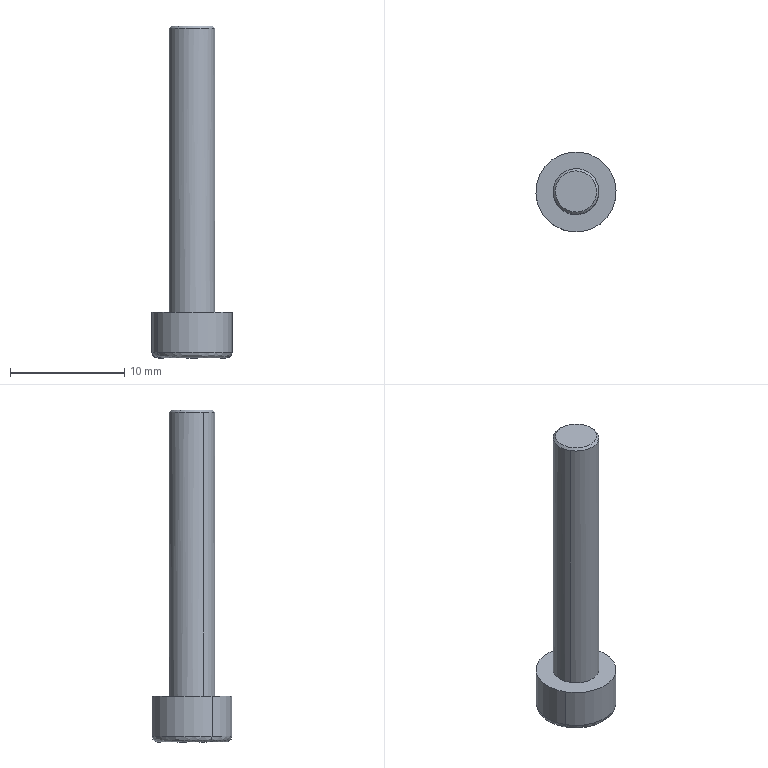Component | SolidWorks | M4X25-5 | 1 solid | 25 faces | box 7 x 7 x 29 mm | volume 449 mm3 | plane 15 | cylinder 4 | cone 4 | spline 2 | commonest cylinder face diameters 4 x2 7 x2 | material Standard Part
STEP:
#1=CARTESIAN_POINT('',(-0.7212,0.5163,-1.24));
#2=VERTEX_POINT('',#1);
#3=CARTESIAN_POINT('',(-0.9599,0.3785,-1.24));
#4=VERTEX_POINT('',#3);
#5=CARTESIAN_POINT('',(-0.8406,0.4474,-1.24));
#6=DIRECTION('',(-0.,-0.,1.));
#7=DIRECTION('',(0.866,0.5,0.));
#8=AXIS2_PLACEMENT_3D('',#5,#6,#7);
#9=CIRCLE('',#8,0.1378);
#10=EDGE_CURVE('',#2,#4,#9,.T.);
#11=ORIENTED_EDGE('',*,*,#10,.F.);
#12=CARTESIAN_POINT('',(-0.7383,0.5065,-1.26));
#13=VERTEX_POINT('',#12);
#14=CARTESIAN_POINT('',(-0.7383,0.5065,-1.24));
#15=DIRECTION('',(-0.5,0.866,-0.));
#16=DIRECTION('',(0.866,0.5,0.));
#17=AXIS2_PLACEMENT_3D('',#14,#15,#16);
#18=CIRCLE('',#17,0.01969);
#19=EDGE_CURVE('',#2,#13,#18,.T.);
#20=ORIENTED_EDGE('',*,*,#19,.T.);
#21=CARTESIAN_POINT('',(-0.9429,0.3884,-1.26));
#22=VERTEX_POINT('',#21);
#23=CARTESIAN_POINT('',(-0.7383,0.5065,-1.26));
#24=CARTESIAN_POINT('',(-0.8564,0.711,-1.26));
#25=CARTESIAN_POINT('',(-1.061,0.5929,-1.26));
#26=CARTESIAN_POINT('',(-0.9429,0.3884,-1.26));
#27=(BOUNDED_CURVE()B_SPLINE_CURVE(3,(#23,#24,#25,#26),.UNSPECIFIED.,.F.,.T.)B_SPLINE_CURVE_WITH_KNOTS((4,4),(0.,1.),.UNSPECIFIED.)CURVE()GEOMETRIC_REPRESENTATION_ITEM()RATIONAL_B_SPLINE_CURVE((1.,0.3333,0.3333,1.))REPRESENTATION_ITEM(''));
#28=EDGE_CURVE('',#13,#22,#27,.T.);
#29=ORIENTED_EDGE('',*,*,#28,.T.);
#30=CARTESIAN_POINT('',(-0.9429,0.3884,-1.24));
#31=DIRECTION('',(0.5,-0.866,0.));
#32=DIRECTION('',(-0.866,-0.5,0.));
#33=AXIS2_PLACEMENT_3D('',#30,#31,#32);
#34=CIRCLE('',#33,0.01969);
#35=EDGE_CURVE('',#4,#22,#34,.T.);
#36=ORIENTED_EDGE('',*,*,#35,.F.);
#37=EDGE_LOOP('',(#11,#20,#29,#36));
#38=FACE_OUTER_BOUND('',#37,.T.);
#39=CARTESIAN_POINT('',(-0.7212,0.5163,-1.24));
#40=CARTESIAN_POINT('',(-0.859,0.755,-1.24));
#41=CARTESIAN_POINT('',(-1.098,0.6172,-1.24));
#42=CARTESIAN_POINT('',(-0.9599,0.3785,-1.24));
#43=CARTESIAN_POINT('',(-0.7212,0.5163,-1.252));
#44=CARTESIAN_POINT('',(-0.859,0.755,-1.252));
#45=CARTESIAN_POINT('',(-1.098,0.6172,-1.252));
#46=CARTESIAN_POINT('',(-0.9599,0.3785,-1.252));
#47=CARTESIAN_POINT('',(-0.7283,0.5122,-1.26));
#48=CARTESIAN_POINT('',(-0.858,0.7368,-1.26));
#49=CARTESIAN_POINT('',(-1.082,0.6071,-1.26));
#50=CARTESIAN_POINT('',(-0.9529,0.3826,-1.26));
#51=CARTESIAN_POINT('',(-0.7383,0.5065,-1.26));
#52=CARTESIAN_POINT('',(-0.8564,0.711,-1.26));
#53=CARTESIAN_POINT('',(-1.061,0.5929,-1.26));
#54=CARTESIAN_POINT('',(-0.9429,0.3884,-1.26));
#55=(BOUNDED_SURFACE()B_SPLINE_SURFACE(3,3,((#39,#40,#41,#42),(#43,#44,#45,#46),(#47,#48,#49,#50),(#51,#52,#53,#54)),.UNSPECIFIED.,.F.,.F.,.F.)B_SPLINE_SURFACE_WITH_KNOTS((4,4),(4,4),(0.,1.),(0.,1.),.UNSPECIFIED.)GEOMETRIC_REPRESENTATION_ITEM()RATIONAL_B_SPLINE_SURFACE(((1.,0.3333,0.3333,1.),(0.8047,0.2682,0.2682,0.8047),(0.8047,0.2682,0.2682,0.8047),(1.,0.3333,0.3333,1.)))REPRESENTATION_ITEM('')SURFACE());
#56=ADVANCED_FACE('',(#38),#55,.T.);
#57=CARTESIAN_POINT('',(-0.8012,0.3792,-0.126));
#58=VERTEX_POINT('',#57);
#59=CARTESIAN_POINT('',(-0.9088,0.408,-0.126));
#60=VERTEX_POINT('',#59);
#61=CARTESIAN_POINT('',(-0.8406,0.4474,-0.126));
#62=DIRECTION('',(0.,0.,-1.));
#63=DIRECTION('',(0.866,0.5,0.));
#64=AXIS2_PLACEMENT_3D('',#61,#62,#63);
#65=CIRCLE('',#64,0.07874);
#66=EDGE_CURVE('',#58,#60,#65,.T.);
#67=ORIENTED_EDGE('',*,*,#66,.T.);
#68=CARTESIAN_POINT('',(-0.9088,0.408,-1.102));
#69=VERTEX_POINT('',#68);
#70=CARTESIAN_POINT('',(-0.9088,0.408,-0.1181));
#71=DIRECTION('',(0.,0.,-1.));
#72=VECTOR('',#71,39.37);
#73=LINE('',#70,#72);
#74=EDGE_CURVE('',#60,#69,#73,.T.);
#75=ORIENTED_EDGE('',*,*,#74,.T.);
#76=CARTESIAN_POINT('',(-0.7724,0.4868,-1.102));
#77=VERTEX_POINT('',#76);
#78=CARTESIAN_POINT('',(-0.8406,0.4474,-1.102));
#79=DIRECTION('',(-0.,-0.,1.));
#80=DIRECTION('',(0.866,0.5,0.));
#81=AXIS2_PLACEMENT_3D('',#78,#79,#80);
#82=CIRCLE('',#81,0.07874);
#83=EDGE_CURVE('',#69,#77,#82,.T.);
#84=ORIENTED_EDGE('',*,*,#83,.T.);
#85=CARTESIAN_POINT('',(-0.7724,0.4868,-0.126));
#86=VERTEX_POINT('',#85);
#87=CARTESIAN_POINT('',(-0.7724,0.4868,-0.1181));
#88=DIRECTION('',(0.,0.,-1.));
#89=VECTOR('',#88,39.37);
#90=LINE('',#87,#89);
#91=EDGE_CURVE('',#86,#77,#90,.T.);
#92=ORIENTED_EDGE('',*,*,#91,.F.);
#93=CARTESIAN_POINT('',(-0.8406,0.4474,-0.126));
#94=DIRECTION('',(0.,0.,-1.));
#95=DIRECTION('',(0.866,0.5,0.));
#96=AXIS2_PLACEMENT_3D('',#93,#94,#95);
#97=CIRCLE('',#96,0.07874);
#98=EDGE_CURVE('',#86,#58,#97,.T.);
#99=ORIENTED_EDGE('',*,*,#98,.T.);
#100=EDGE_LOOP('',(#67,#75,#84,#92,#99));
#101=FACE_OUTER_BOUND('',#100,.T.);
#102=CARTESIAN_POINT('',(-0.8406,0.4474,-0.1181));
#103=DIRECTION('',(0.,0.,-1.));
#104=DIRECTION('',(0.866,0.5,0.));
#105=AXIS2_PLACEMENT_3D('',#102,#103,#104);
#106=CYLINDRICAL_SURFACE('',#105,0.07874);
#107=ADVANCED_FACE('',(#101),#106,.T.);
#108=CARTESIAN_POINT('',(-0.876,0.5088,-0.1181));
#109=VERTEX_POINT('',#108);
#110=CARTESIAN_POINT('',(-0.8051,0.386,-0.1181));
#111=VERTEX_POINT('',#110);
#112=CARTESIAN_POINT('',(-0.8406,0.4474,-0.1181));
#113=DIRECTION('',(-0.,0.,-1.));
#114=DIRECTION('',(-0.5,0.866,0.));
#115=AXIS2_PLACEMENT_3D('',#112,#113,#114);
#116=CIRCLE('',#115,0.07087);
#117=EDGE_CURVE('',#109,#111,#116,.T.);
#118=ORIENTED_EDGE('',*,*,#117,.T.);
#119=CARTESIAN_POINT('',(-0.8012,0.3792,-0.126));
#120=DIRECTION('',(0.3536,-0.6124,-0.7071));
#121=VECTOR('',#120,39.37);
#122=LINE('',#119,#121);
#123=EDGE_CURVE('',#111,#58,#122,.T.);
#124=ORIENTED_EDGE('',*,*,#123,.T.);
#125=ORIENTED_EDGE('',*,*,#98,.F.);
#126=CARTESIAN_POINT('',(-0.88,0.5156,-0.126));
#127=VERTEX_POINT('',#126);
#128=CARTESIAN_POINT('',(-0.8406,0.4474,-0.126));
#129=DIRECTION('',(0.,0.,-1.));
#130=DIRECTION('',(0.866,0.5,0.));
#131=AXIS2_PLACEMENT_3D('',#128,#129,#130);
#132=CIRCLE('',#131,0.07874);
#133=EDGE_CURVE('',#127,#86,#132,.T.);
#134=ORIENTED_EDGE('',*,*,#133,.F.);
#135=CARTESIAN_POINT('',(-0.88,0.5156,-0.126));
#136=DIRECTION('',(-0.3536,0.6124,-0.7071));
#137=VECTOR('',#136,39.37);
#138=LINE('',#135,#137);
#139=EDGE_CURVE('',#109,#127,#138,.T.);
#140=ORIENTED_EDGE('',*,*,#139,.F.);
#141=EDGE_LOOP('',(#118,#124,#125,#134,#140));
#142=FACE_OUTER_BOUND('',#141,.T.);
#143=CARTESIAN_POINT('',(-0.8406,0.4474,-0.126));
#144=DIRECTION('',(-0.,0.,-1.));
#145=DIRECTION('',(-0.5,0.866,0.));
#146=AXIS2_PLACEMENT_3D('',#143,#144,#145);
#147=CONICAL_SURFACE('',#146,0.07874,0.7854);
#148=ADVANCED_FACE('',(#142),#147,.T.);
#149=CARTESIAN_POINT('',(-0.9599,0.3785,-1.102));
#150=VERTEX_POINT('',#149);
#151=CARTESIAN_POINT('',(-0.7212,0.5163,-1.102));
#152=VERTEX_POINT('',#151);
#153=CARTESIAN_POINT('',(-0.8406,0.4474,-1.102));
#154=DIRECTION('',(-0.,-0.,1.));
#155=DIRECTION('',(0.866,0.5,0.));
#156=AXIS2_PLACEMENT_3D('',#153,#154,#155);
#157=CIRCLE('',#156,0.1378);
#158=EDGE_CURVE('',#150,#152,#157,.T.);
#159=ORIENTED_EDGE('',*,*,#158,.F.);
#160=CARTESIAN_POINT('',(-0.9599,0.3785,-1.102));
#161=DIRECTION('',(0.,0.,-1.));
#162=VECTOR('',#161,39.37);
#163=LINE('',#160,#162);
#164=EDGE_CURVE('',#150,#4,#163,.T.);
#165=ORIENTED_EDGE('',*,*,#164,.T.);
#166=CARTESIAN_POINT('',(-0.8406,0.4474,-1.24));
#167=DIRECTION('',(-0.,-0.,1.));
#168=DIRECTION('',(0.866,0.5,0.));
#169=AXIS2_PLACEMENT_3D('',#166,#167,#168);
#170=CIRCLE('',#169,0.1378);
#171=EDGE_CURVE('',#4,#2,#170,.T.);
#172=ORIENTED_EDGE('',*,*,#171,.T.);
#173=CARTESIAN_POINT('',(-0.7212,0.5163,-1.102));
#174=DIRECTION('',(0.,0.,-1.));
#175=VECTOR('',#174,39.37);
#176=LINE('',#173,#175);
#177=EDGE_CURVE('',#152,#2,#176,.T.);
#178=ORIENTED_EDGE('',*,*,#177,.F.);
#179=EDGE_LOOP('',(#159,#165,#172,#178));
#180=FACE_OUTER_BOUND('',#179,.T.);
#181=CARTESIAN_POINT('',(-0.8406,0.4474,-1.102));
#182=DIRECTION('',(0.,0.,-1.));
#183=DIRECTION('',(0.866,0.5,0.));
#184=AXIS2_PLACEMENT_3D('',#181,#182,#183);
#185=CYLINDRICAL_SURFACE('',#184,0.1378);
#186=ADVANCED_FACE('',(#180),#185,.T.);
#187=CARTESIAN_POINT('',(-0.8406,0.4474,-1.147));
#188=VERTEX_POINT('',#187);
#189=CARTESIAN_POINT('',(-0.7894,0.4769,-1.181));
#190=VERTEX_POINT('',#189);
#191=CARTESIAN_POINT('',(-0.7894,0.4769,-1.181));
#192=DIRECTION('',(0.75,0.433,-0.5));
#193=VECTOR('',#192,39.37);
#194=LINE('',#191,#193);
#195=EDGE_CURVE('',#188,#190,#194,.T.);
#196=ORIENTED_EDGE('',*,*,#195,.F.);
#197=CARTESIAN_POINT('',(-0.8917,0.4179,-1.181));
#198=VERTEX_POINT('',#197);
#199=CARTESIAN_POINT('',(-0.8917,0.4179,-1.181));
#200=DIRECTION('',(-0.75,-0.433,-0.5));
#201=VECTOR('',#200,39.37);
#202=LINE('',#199,#201);
#203=EDGE_CURVE('',#188,#198,#202,.T.);
#204=ORIENTED_EDGE('',*,*,#203,.T.);
#205=CARTESIAN_POINT('',(-0.8996,0.4474,-1.181));
#206=VERTEX_POINT('',#205);
#207=CARTESIAN_POINT('',(-0.8406,0.4474,-1.181));
#208=DIRECTION('',(-0.,-0.,1.));
#209=DIRECTION('',(0.866,0.5,0.));
#210=AXIS2_PLACEMENT_3D('',#207,#208,#209);
#211=CIRCLE('',#210,0.05906);
#212=EDGE_CURVE('',#206,#198,#211,.T.);
#213=ORIENTED_EDGE('',*,*,#212,.F.);
#214=CARTESIAN_POINT('',(-0.8701,0.4986,-1.181));
#215=VERTEX_POINT('',#214);
#216=CARTESIAN_POINT('',(-0.8406,0.4474,-1.181));
#217=DIRECTION('',(0.,0.,-1.));
#218=DIRECTION('',(0.866,0.5,0.));
#219=AXIS2_PLACEMENT_3D('',#216,#217,#218);
#220=CIRCLE('',#219,0.05906);
#221=EDGE_CURVE('',#206,#215,#220,.T.);
#222=ORIENTED_EDGE('',*,*,#221,.T.);
#223=CARTESIAN_POINT('',(-0.8111,0.4986,-1.181));
#224=VERTEX_POINT('',#223);
#225=CARTESIAN_POINT('',(-0.8406,0.4474,-1.181));
#226=DIRECTION('',(-0.,-0.,1.));
#227=DIRECTION('',(0.866,0.5,0.));
#228=AXIS2_PLACEMENT_3D('',#225,#226,#227);
#229=CIRCLE('',#228,0.05906);
#230=EDGE_CURVE('',#224,#215,#229,.T.);
#231=ORIENTED_EDGE('',*,*,#230,.F.);
#232=CARTESIAN_POINT('',(-0.8406,0.4474,-1.181));
#233=DIRECTION('',(-0.,-0.,1.));
#234=DIRECTION('',(0.866,0.5,0.));
#235=AXIS2_PLACEMENT_3D('',#232,#233,#234);
#236=CIRCLE('',#235,0.05906);
#237=EDGE_CURVE('',#190,#224,#236,.T.);
#238=ORIENTED_EDGE('',*,*,#237,.F.);
#239=EDGE_LOOP('',(#196,#204,#213,#222,#231,#238));
#240=FACE_OUTER_BOUND('',#239,.T.);
#241=CARTESIAN_POINT('',(-0.8406,0.4474,-1.181));
#242=DIRECTION('',(0.,0.,-1.));
#243=DIRECTION('',(0.866,0.5,0.));
#244=AXIS2_PLACEMENT_3D('',#241,#242,#243);
#245=CONICAL_SURFACE('',#244,0.05906,1.047);
#246=ADVANCED_FACE('',(#240),#245,.F.);
#247=ORIENTED_EDGE('',*,*,#74,.F.);
#248=CARTESIAN_POINT('',(-0.8406,0.4474,-0.126));
#249=DIRECTION('',(0.,0.,-1.));
#250=DIRECTION('',(0.866,0.5,0.));
#251=AXIS2_PLACEMENT_3D('',#248,#249,#250);
#252=CIRCLE('',#251,0.07874);
#253=EDGE_CURVE('',#60,#127,#252,.T.);
#254=ORIENTED_EDGE('',*,*,#253,.T.);
#255=ORIENTED_EDGE('',*,*,#133,.T.);
#256=ORIENTED_EDGE('',*,*,#91,.T.);
#257=CARTESIAN_POINT('',(-0.8406,0.4474,-1.102));
#258=DIRECTION('',(-0.,-0.,1.));
#259=DIRECTION('',(0.866,0.5,0.));
#260=AXIS2_PLACEMENT_3D('',#257,#258,#259);
#261=CIRCLE('',#260,0.07874);
#262=EDGE_CURVE('',#77,#69,#261,.T.);
#263=ORIENTED_EDGE('',*,*,#262,.T.);
#264=EDGE_LOOP('',(#247,#254,#255,#256,#263));
#265=FACE_OUTER_BOUND('',#264,.T.);
#266=CARTESIAN_POINT('',(-0.8406,0.4474,-0.1181));
#267=DIRECTION('',(0.,0.,-1.));
#268=DIRECTION('',(0.866,0.5,0.));
#269=AXIS2_PLACEMENT_3D('',#266,#267,#268);
#270=CYLINDRICAL_SURFACE('',#269,0.07874);
#271=ADVANCED_FACE('',(#265),#270,.T.);
#272=ORIENTED_EDGE('',*,*,#262,.F.);
#273=ORIENTED_EDGE('',*,*,#83,.F.);
#274=EDGE_LOOP('',(#272,#273));
#275=FACE_BOUND('',#274,.T.);
#276=CARTESIAN_POINT('',(-0.8406,0.4474,-1.102));
#277=DIRECTION('',(-0.,-0.,1.));
#278=DIRECTION('',(0.866,0.5,0.));
#279=AXIS2_PLACEMENT_3D('',#276,#277,#278);
#280=CIRCLE('',#279,0.1378);
#281=EDGE_CURVE('',#152,#150,#280,.T.);
#282=ORIENTED_EDGE('',*,*,#281,.T.);
#283=ORIENTED_EDGE('',*,*,#158,.T.);
#284=EDGE_LOOP('',(#282,#283));
#285=FACE_OUTER_BOUND('',#284,.T.);
#286=CARTESIAN_POINT('',(-0.8406,0.4474,-1.102));
#287=DIRECTION('',(-0.,-0.,1.));
#288=DIRECTION('',(-0.866,-0.5,-0.));
#289=AXIS2_PLACEMENT_3D('',#286,#287,#288);
#290=PLANE('',#289);
#291=ADVANCED_FACE('',(#275,#285),#290,.T.);
#292=ORIENTED_EDGE('',*,*,#123,.F.);
#293=CARTESIAN_POINT('',(-0.8406,0.4474,-0.1181));
#294=DIRECTION('',(-0.,0.,-1.));
#295=DIRECTION('',(-0.5,0.866,0.));
#296=AXIS2_PLACEMENT_3D('',#293,#294,#295);
#297=CIRCLE('',#296,0.07087);
#298=EDGE_CURVE('',#111,#109,#297,.T.);
#299=ORIENTED_EDGE('',*,*,#298,.T.);
#300=ORIENTED_EDGE('',*,*,#139,.T.);
#301=ORIENTED_EDGE('',*,*,#253,.F.);
#302=ORIENTED_EDGE('',*,*,#66,.F.);
#303=EDGE_LOOP('',(#292,#299,#300,#301,#302));
#304=FACE_OUTER_BOUND('',#303,.T.);
#305=CARTESIAN_POINT('',(-0.8406,0.4474,-0.126));
#306=DIRECTION('',(-0.,0.,-1.));
#307=DIRECTION('',(-0.5,0.866,0.));
#308=AXIS2_PLACEMENT_3D('',#305,#306,#307);
#309=CONICAL_SURFACE('',#308,0.07874,0.7854);
#310=ADVANCED_FACE('',(#304),#309,.T.);
#311=ORIENTED_EDGE('',*,*,#164,.F.);
#312=ORIENTED_EDGE('',*,*,#281,.F.);
#313=ORIENTED_EDGE('',*,*,#177,.T.);
#314=ORIENTED_EDGE('',*,*,#10,.T.);
#315=EDGE_LOOP('',(#311,#312,#313,#314));
#316=FACE_OUTER_BOUND('',#315,.T.);
#317=CARTESIAN_POINT('',(-0.8406,0.4474,-1.102));
#318=DIRECTION('',(0.,0.,-1.));
#319=DIRECTION('',(0.866,0.5,0.));
#320=AXIS2_PLACEMENT_3D('',#317,#318,#319);
#321=CYLINDRICAL_SURFACE('',#320,0.1378);
#322=ADVANCED_FACE('',(#316),#321,.T.);
#323=ORIENTED_EDGE('',*,*,#117,.F.);
#324=ORIENTED_EDGE('',*,*,#298,.F.);
#325=EDGE_LOOP('',(#323,#324));
#326=FACE_OUTER_BOUND('',#325,.T.);
#327=CARTESIAN_POINT('',(-0.8406,0.4474,-0.1181));
#328=DIRECTION('',(-0.,-0.,1.));
#329=DIRECTION('',(-0.866,-0.5,-0.));
#330=AXIS2_PLACEMENT_3D('',#327,#328,#329);
#331=PLANE('',#330);
#332=ADVANCED_FACE('',(#326),#331,.T.);
#333=ORIENTED_EDGE('',*,*,#19,.F.);
#334=ORIENTED_EDGE('',*,*,#171,.F.);
#335=ORIENTED_EDGE('',*,*,#35,.T.);
#336=CARTESIAN_POINT('',(-0.9429,0.3884,-1.26));
#337=CARTESIAN_POINT('',(-0.8248,0.1838,-1.26));
#338=CARTESIAN_POINT('',(-0.6202,0.3019,-1.26));
#339=CARTESIAN_POINT('',(-0.7383,0.5065,-1.26));
#340=(BOUNDED_CURVE()B_SPLINE_CURVE(3,(#336,#337,#338,#339),.UNSPECIFIED.,.F.,.T.)B_SPLINE_CURVE_WITH_KNOTS((4,4),(0.,1.),.UNSPECIFIED.)CURVE()GEOMETRIC_REPRESENTATION_ITEM()RATIONAL_B_SPLINE_CURVE((1.,0.3333,0.3333,1.))REPRESENTATION_ITEM(''));
#341=EDGE_CURVE('',#22,#13,#340,.T.);
#342=ORIENTED_EDGE('',*,*,#341,.T.);
#343=EDGE_LOOP('',(#333,#334,#335,#342));
#344=FACE_OUTER_BOUND('',#343,.T.);
#345=CARTESIAN_POINT('',(-0.9599,0.3785,-1.24));
#346=CARTESIAN_POINT('',(-0.8221,0.1398,-1.24));
#347=CARTESIAN_POINT('',(-0.5835,0.2776,-1.24));
#348=CARTESIAN_POINT('',(-0.7212,0.5163,-1.24));
#349=CARTESIAN_POINT('',(-0.9599,0.3785,-1.252));
#350=CARTESIAN_POINT('',(-0.8221,0.1398,-1.252));
#351=CARTESIAN_POINT('',(-0.5835,0.2776,-1.252));
#352=CARTESIAN_POINT('',(-0.7212,0.5163,-1.252));
#353=CARTESIAN_POINT('',(-0.9529,0.3826,-1.26));
#354=CARTESIAN_POINT('',(-0.8232,0.158,-1.26));
#355=CARTESIAN_POINT('',(-0.5987,0.2877,-1.26));
#356=CARTESIAN_POINT('',(-0.7283,0.5122,-1.26));
#357=CARTESIAN_POINT('',(-0.9429,0.3884,-1.26));
#358=CARTESIAN_POINT('',(-0.8248,0.1838,-1.26));
#359=CARTESIAN_POINT('',(-0.6202,0.3019,-1.26));
#360=CARTESIAN_POINT('',(-0.7383,0.5065,-1.26));
#361=(BOUNDED_SURFACE()B_SPLINE_SURFACE(3,3,((#345,#346,#347,#348),(#349,#350,#351,#352),(#353,#354,#355,#356),(#357,#358,#359,#360)),.UNSPECIFIED.,.F.,.F.,.F.)B_SPLINE_SURFACE_WITH_KNOTS((4,4),(4,4),(0.,1.),(0.,1.),.UNSPECIFIED.)GEOMETRIC_REPRESENTATION_ITEM()RATIONAL_B_SPLINE_SURFACE(((1.,0.3333,0.3333,1.),(0.8047,0.2682,0.2682,0.8047),(0.8047,0.2682,0.2682,0.8047),(1.,0.3333,0.3333,1.)))REPRESENTATION_ITEM('')SURFACE());
#362=ADVANCED_FACE('',(#344),#361,.T.);
#363=CARTESIAN_POINT('',(-0.8406,0.3792,-1.26));
#364=VERTEX_POINT('',#363);
#365=CARTESIAN_POINT('',(-0.8996,0.4133,-1.26));
#366=VERTEX_POINT('',#365);
#367=CARTESIAN_POINT('',(-0.8996,0.4133,-1.26));
#368=DIRECTION('',(-0.866,0.5,-0.));
#369=VECTOR('',#368,39.37);
#370=LINE('',#367,#369);
#371=EDGE_CURVE('',#364,#366,#370,.T.);
#372=ORIENTED_EDGE('',*,*,#371,.F.);
#373=CARTESIAN_POINT('',(-0.7815,0.4133,-1.26));
#374=VERTEX_POINT('',#373);
#375=CARTESIAN_POINT('',(-0.8406,0.3792,-1.26));
#376=DIRECTION('',(-0.866,-0.5,-0.));
#377=VECTOR('',#376,39.37);
#378=LINE('',#375,#377);
#379=EDGE_CURVE('',#374,#364,#378,.T.);
#380=ORIENTED_EDGE('',*,*,#379,.F.);
#381=CARTESIAN_POINT('',(-0.7815,0.4815,-1.26));
#382=VERTEX_POINT('',#381);
#383=CARTESIAN_POINT('',(-0.7815,0.4133,-1.26));
#384=DIRECTION('',(-0.,-1.,-0.));
#385=VECTOR('',#384,39.37);
#386=LINE('',#383,#385);
#387=EDGE_CURVE('',#382,#374,#386,.T.);
#388=ORIENTED_EDGE('',*,*,#387,.F.);
#389=CARTESIAN_POINT('',(-0.8406,0.5156,-1.26));
#390=VERTEX_POINT('',#389);
#391=CARTESIAN_POINT('',(-0.7815,0.4815,-1.26));
#392=DIRECTION('',(0.866,-0.5,0.));
#393=VECTOR('',#392,39.37);
#394=LINE('',#391,#393);
#395=EDGE_CURVE('',#390,#382,#394,.T.);
#396=ORIENTED_EDGE('',*,*,#395,.F.);
#397=CARTESIAN_POINT('',(-0.8996,0.4815,-1.26));
#398=VERTEX_POINT('',#397);
#399=CARTESIAN_POINT('',(-0.8406,0.5156,-1.26));
#400=DIRECTION('',(0.866,0.5,0.));
#401=VECTOR('',#400,39.37);
#402=LINE('',#399,#401);
#403=EDGE_CURVE('',#398,#390,#402,.T.);
#404=ORIENTED_EDGE('',*,*,#403,.F.);
#405=CARTESIAN_POINT('',(-0.8996,0.4133,-1.26));
#406=DIRECTION('',(0.,1.,0.));
#407=VECTOR('',#406,39.37);
#408=LINE('',#405,#407);
#409=EDGE_CURVE('',#366,#398,#408,.T.);
#410=ORIENTED_EDGE('',*,*,#409,.F.);
#411=EDGE_LOOP('',(#372,#380,#388,#396,#404,#410));
#412=FACE_BOUND('',#411,.T.);
#413=ORIENTED_EDGE('',*,*,#341,.F.);
#414=ORIENTED_EDGE('',*,*,#28,.F.);
#415=EDGE_LOOP('',(#413,#414));
#416=FACE_OUTER_BOUND('',#415,.T.);
#417=CARTESIAN_POINT('',(-0.8406,0.4474,-1.26));
#418=DIRECTION('',(-0.,-0.,1.));
#419=DIRECTION('',(-0.866,-0.5,-0.));
#420=AXIS2_PLACEMENT_3D('',#417,#418,#419);
#421=PLANE('',#420);
#422=ADVANCED_FACE('',(#412,#416),#421,.F.);
#423=CARTESIAN_POINT('',(-0.8996,0.4133,-1.181));
#424=VERTEX_POINT('',#423);
#425=CARTESIAN_POINT('',(-0.8996,0.4815,-1.181));
#426=DIRECTION('',(-0.,-1.,-0.));
#427=VECTOR('',#426,39.37);
#428=LINE('',#425,#427);
#429=EDGE_CURVE('',#206,#424,#428,.T.);
#430=ORIENTED_EDGE('',*,*,#429,.T.);
#431=CARTESIAN_POINT('',(-0.8996,0.4133,-1.181));
#432=DIRECTION('',(0.,0.,-1.));
#433=VECTOR('',#432,39.37);
#434=LINE('',#431,#433);
#435=EDGE_CURVE('',#424,#366,#434,.T.);
#436=ORIENTED_EDGE('',*,*,#435,.T.);
#437=ORIENTED_EDGE('',*,*,#409,.T.);
#438=CARTESIAN_POINT('',(-0.8996,0.4815,-1.181));
#439=VERTEX_POINT('',#438);
#440=CARTESIAN_POINT('',(-0.8996,0.4815,-1.181));
#441=DIRECTION('',(-0.,-0.,1.));
#442=VECTOR('',#441,39.37);
#443=LINE('',#440,#442);
#444=EDGE_CURVE('',#398,#439,#443,.T.);
#445=ORIENTED_EDGE('',*,*,#444,.T.);
#446=CARTESIAN_POINT('',(-0.8996,0.4815,-1.181));
#447=DIRECTION('',(-0.,-1.,-0.));
#448=VECTOR('',#447,39.37);
#449=LINE('',#446,#448);
#450=EDGE_CURVE('',#439,#206,#449,.T.);
#451=ORIENTED_EDGE('',*,*,#450,.T.);
#452=EDGE_LOOP('',(#430,#436,#437,#445,#451));
#453=FACE_OUTER_BOUND('',#452,.T.);
#454=CARTESIAN_POINT('',(-0.8996,0.4815,-1.181));
#455=DIRECTION('',(1.,-0.,0.));
#456=DIRECTION('',(0.,1.,0.));
#457=AXIS2_PLACEMENT_3D('',#454,#455,#456);
#458=PLANE('',#457);
#459=ADVANCED_FACE('',(#453),#458,.T.);
#460=CARTESIAN_POINT('',(-0.8701,0.3963,-1.181));
#461=VERTEX_POINT('',#460);
#462=CARTESIAN_POINT('',(-0.8406,0.3792,-1.181));
#463=VERTEX_POINT('',#462);
#464=CARTESIAN_POINT('',(-0.8996,0.4133,-1.181));
#465=DIRECTION('',(0.866,-0.5,0.));
#466=VECTOR('',#465,39.37);
#467=LINE('',#464,#466);
#468=EDGE_CURVE('',#461,#463,#467,.T.);
#469=ORIENTED_EDGE('',*,*,#468,.T.);
#470=CARTESIAN_POINT('',(-0.8406,0.3792,-1.181));
#471=DIRECTION('',(0.,0.,-1.));
#472=VECTOR('',#471,39.37);
#473=LINE('',#470,#472);
#474=EDGE_CURVE('',#463,#364,#473,.T.);
#475=ORIENTED_EDGE('',*,*,#474,.T.);
#476=ORIENTED_EDGE('',*,*,#371,.T.);
#477=ORIENTED_EDGE('',*,*,#435,.F.);
#478=CARTESIAN_POINT('',(-0.8996,0.4133,-1.181));
#479=DIRECTION('',(0.866,-0.5,0.));
#480=VECTOR('',#479,39.37);
#481=LINE('',#478,#480);
#482=EDGE_CURVE('',#424,#461,#481,.T.);
#483=ORIENTED_EDGE('',*,*,#482,.T.);
#484=EDGE_LOOP('',(#469,#475,#476,#477,#483));
#485=FACE_OUTER_BOUND('',#484,.T.);
#486=CARTESIAN_POINT('',(-0.8996,0.4133,-1.181));
#487=DIRECTION('',(0.5,0.866,0.));
#488=DIRECTION('',(-0.866,0.5,-0.));
#489=AXIS2_PLACEMENT_3D('',#486,#487,#488);
#490=PLANE('',#489);
#491=ADVANCED_FACE('',(#485),#490,.T.);
#492=ORIENTED_EDGE('',*,*,#482,.F.);
#493=ORIENTED_EDGE('',*,*,#429,.F.);
#494=ORIENTED_EDGE('',*,*,#212,.T.);
#495=CARTESIAN_POINT('',(-0.8406,0.4474,-1.181));
#496=DIRECTION('',(-0.,-0.,1.));
#497=DIRECTION('',(0.866,0.5,0.));
#498=AXIS2_PLACEMENT_3D('',#495,#496,#497);
#499=CIRCLE('',#498,0.05906);
#500=EDGE_CURVE('',#198,#461,#499,.T.);
#501=ORIENTED_EDGE('',*,*,#500,.T.);
#502=EDGE_LOOP('',(#492,#493,#494,#501));
#503=FACE_OUTER_BOUND('',#502,.T.);
#504=CARTESIAN_POINT('',(-0.8996,0.3451,-1.181));
#505=DIRECTION('',(-0.,-0.,1.));
#506=DIRECTION('',(-0.866,-0.5,-0.));
#507=AXIS2_PLACEMENT_3D('',#504,#505,#506);
#508=PLANE('',#507);
#509=ADVANCED_FACE('',(#503),#508,.F.);
#510=ORIENTED_EDGE('',*,*,#450,.F.);
#511=CARTESIAN_POINT('',(-0.9587,0.4474,-1.181));
#512=DIRECTION('',(-0.866,-0.5,-0.));
#513=VECTOR('',#512,39.37);
#514=LINE('',#511,#513);
#515=EDGE_CURVE('',#215,#439,#514,.T.);
#516=ORIENTED_EDGE('',*,*,#515,.F.);
#517=ORIENTED_EDGE('',*,*,#221,.F.);
#518=EDGE_LOOP('',(#510,#516,#517));
#519=FACE_OUTER_BOUND('',#518,.T.);
#520=CARTESIAN_POINT('',(-0.8996,0.3451,-1.181));
#521=DIRECTION('',(-0.,-0.,1.));
#522=DIRECTION('',(-0.866,-0.5,-0.));
#523=AXIS2_PLACEMENT_3D('',#520,#521,#522);
#524=PLANE('',#523);
#525=ADVANCED_FACE('',(#519),#524,.F.);
#526=ORIENTED_EDGE('',*,*,#515,.T.);
#527=ORIENTED_EDGE('',*,*,#444,.F.);
#528=ORIENTED_EDGE('',*,*,#403,.T.);
#529=CARTESIAN_POINT('',(-0.8406,0.5156,-1.181));
#530=VERTEX_POINT('',#529);
#531=CARTESIAN_POINT('',(-0.8406,0.5156,-1.181));
#532=DIRECTION('',(-0.,-0.,1.));
#533=VECTOR('',#532,39.37);
#534=LINE('',#531,#533);
#535=EDGE_CURVE('',#390,#530,#534,.T.);
#536=ORIENTED_EDGE('',*,*,#535,.T.);
#537=CARTESIAN_POINT('',(-0.8406,0.5156,-1.181));
#538=DIRECTION('',(-0.866,-0.5,-0.));
#539=VECTOR('',#538,39.37);
#540=LINE('',#537,#539);
#541=EDGE_CURVE('',#530,#215,#540,.T.);
#542=ORIENTED_EDGE('',*,*,#541,.T.);
#543=EDGE_LOOP('',(#526,#527,#528,#536,#542));
#544=FACE_OUTER_BOUND('',#543,.T.);
#545=CARTESIAN_POINT('',(-0.8406,0.5156,-1.181));
#546=DIRECTION('',(0.5,-0.866,0.));
#547=DIRECTION('',(0.866,0.5,0.));
#548=AXIS2_PLACEMENT_3D('',#545,#546,#547);
#549=PLANE('',#548);
#550=ADVANCED_FACE('',(#544),#549,.T.);
#551=CARTESIAN_POINT('',(-0.8111,0.3963,-1.181));
#552=VERTEX_POINT('',#551);
#553=CARTESIAN_POINT('',(-0.7815,0.4133,-1.181));
#554=VERTEX_POINT('',#553);
#555=CARTESIAN_POINT('',(-0.8406,0.3792,-1.181));
#556=DIRECTION('',(0.866,0.5,0.));
#557=VECTOR('',#556,39.37);
#558=LINE('',#555,#557);
#559=EDGE_CURVE('',#552,#554,#558,.T.);
#560=ORIENTED_EDGE('',*,*,#559,.T.);
#561=CARTESIAN_POINT('',(-0.7815,0.4133,-1.181));
#562=DIRECTION('',(0.,0.,-1.));
#563=VECTOR('',#562,39.37);
#564=LINE('',#561,#563);
#565=EDGE_CURVE('',#554,#374,#564,.T.);
#566=ORIENTED_EDGE('',*,*,#565,.T.);
#567=ORIENTED_EDGE('',*,*,#379,.T.);
#568=ORIENTED_EDGE('',*,*,#474,.F.);
#569=CARTESIAN_POINT('',(-0.8406,0.3792,-1.181));
#570=DIRECTION('',(0.866,0.5,0.));
#571=VECTOR('',#570,39.37);
#572=LINE('',#569,#571);
#573=EDGE_CURVE('',#463,#552,#572,.T.);
#574=ORIENTED_EDGE('',*,*,#573,.T.);
#575=EDGE_LOOP('',(#560,#566,#567,#568,#574));
#576=FACE_OUTER_BOUND('',#575,.T.);
#577=CARTESIAN_POINT('',(-0.8406,0.3792,-1.181));
#578=DIRECTION('',(-0.5,0.866,-0.));
#579=DIRECTION('',(-0.866,-0.5,-0.));
#580=AXIS2_PLACEMENT_3D('',#577,#578,#579);
#581=PLANE('',#580);
#582=ADVANCED_FACE('',(#576),#581,.T.);
#583=ORIENTED_EDGE('',*,*,#573,.F.);
#584=ORIENTED_EDGE('',*,*,#468,.F.);
#585=CARTESIAN_POINT('',(-0.8406,0.4474,-1.181));
#586=DIRECTION('',(0.,0.,-1.));
#587=DIRECTION('',(0.866,0.5,0.));
#588=AXIS2_PLACEMENT_3D('',#585,#586,#587);
#589=CIRCLE('',#588,0.05906);
#590=EDGE_CURVE('',#552,#461,#589,.T.);
#591=ORIENTED_EDGE('',*,*,#590,.F.);
#592=EDGE_LOOP('',(#583,#584,#591));
#593=FACE_OUTER_BOUND('',#592,.T.);
#594=CARTESIAN_POINT('',(-0.8996,0.3451,-1.181));
#595=DIRECTION('',(-0.,-0.,1.));
#596=DIRECTION('',(-0.866,-0.5,-0.));
#597=AXIS2_PLACEMENT_3D('',#594,#595,#596);
#598=PLANE('',#597);
#599=ADVANCED_FACE('',(#593),#598,.F.);
#600=ORIENTED_EDGE('',*,*,#203,.F.);
#601=ORIENTED_EDGE('',*,*,#195,.T.);
#602=CARTESIAN_POINT('',(-0.7815,0.4474,-1.181));
#603=VERTEX_POINT('',#602);
#604=CARTESIAN_POINT('',(-0.8406,0.4474,-1.181));
#605=DIRECTION('',(-0.,-0.,1.));
#606=DIRECTION('',(0.866,0.5,0.));
#607=AXIS2_PLACEMENT_3D('',#604,#605,#606);
#608=CIRCLE('',#607,0.05906);
#609=EDGE_CURVE('',#603,#190,#608,.T.);
#610=ORIENTED_EDGE('',*,*,#609,.F.);
#611=CARTESIAN_POINT('',(-0.8406,0.4474,-1.181));
#612=DIRECTION('',(0.,0.,-1.));
#613=DIRECTION('',(0.866,0.5,0.));
#614=AXIS2_PLACEMENT_3D('',#611,#612,#613);
#615=CIRCLE('',#614,0.05906);
#616=EDGE_CURVE('',#603,#552,#615,.T.);
#617=ORIENTED_EDGE('',*,*,#616,.T.);
#618=ORIENTED_EDGE('',*,*,#590,.T.);
#619=ORIENTED_EDGE('',*,*,#500,.F.);
#620=EDGE_LOOP('',(#600,#601,#610,#617,#618,#619));
#621=FACE_OUTER_BOUND('',#620,.T.);
#622=CARTESIAN_POINT('',(-0.8406,0.4474,-1.181));
#623=DIRECTION('',(0.,0.,-1.));
#624=DIRECTION('',(0.866,0.5,0.));
#625=AXIS2_PLACEMENT_3D('',#622,#623,#624);
#626=CONICAL_SURFACE('',#625,0.05906,1.047);
#627=ADVANCED_FACE('',(#621),#626,.F.);
#628=ORIENTED_EDGE('',*,*,#541,.F.);
#629=CARTESIAN_POINT('',(-0.8111,0.4986,-1.181));
#630=DIRECTION('',(-0.866,0.5,-0.));
#631=VECTOR('',#630,39.37);
#632=LINE('',#629,#631);
#633=EDGE_CURVE('',#224,#530,#632,.T.);
#634=ORIENTED_EDGE('',*,*,#633,.F.);
#635=ORIENTED_EDGE('',*,*,#230,.T.);
#636=EDGE_LOOP('',(#628,#634,#635));
#637=FACE_OUTER_BOUND('',#636,.T.);
#638=CARTESIAN_POINT('',(-0.8996,0.3451,-1.181));
#639=DIRECTION('',(-0.,-0.,1.));
#640=DIRECTION('',(-0.866,-0.5,-0.));
#641=AXIS2_PLACEMENT_3D('',#638,#639,#640);
#642=PLANE('',#641);
#643=ADVANCED_FACE('',(#637),#642,.F.);
#644=ORIENTED_EDGE('',*,*,#633,.T.);
#645=ORIENTED_EDGE('',*,*,#535,.F.);
#646=ORIENTED_EDGE('',*,*,#395,.T.);
#647=CARTESIAN_POINT('',(-0.7815,0.4815,-1.181));
#648=VERTEX_POINT('',#647);
#649=CARTESIAN_POINT('',(-0.7815,0.4815,-1.181));
#650=DIRECTION('',(-0.,-0.,1.));
#651=VECTOR('',#650,39.37);
#652=LINE('',#649,#651);
#653=EDGE_CURVE('',#382,#648,#652,.T.);
#654=ORIENTED_EDGE('',*,*,#653,.T.);
#655=CARTESIAN_POINT('',(-0.7815,0.4815,-1.181));
#656=DIRECTION('',(-0.866,0.5,-0.));
#657=VECTOR('',#656,39.37);
#658=LINE('',#655,#657);
#659=EDGE_CURVE('',#648,#224,#658,.T.);
#660=ORIENTED_EDGE('',*,*,#659,.T.);
#661=EDGE_LOOP('',(#644,#645,#646,#654,#660));
#662=FACE_OUTER_BOUND('',#661,.T.);
#663=CARTESIAN_POINT('',(-0.7815,0.4815,-1.181));
#664=DIRECTION('',(-0.5,-0.866,-0.));
#665=DIRECTION('',(0.866,-0.5,0.));
#666=AXIS2_PLACEMENT_3D('',#663,#664,#665);
#667=PLANE('',#666);
#668=ADVANCED_FACE('',(#662),#667,.T.);
#669=CARTESIAN_POINT('',(-0.7815,0.4133,-1.181));
#670=DIRECTION('',(0.,1.,0.));
#671=VECTOR('',#670,39.37);
#672=LINE('',#669,#671);
#673=EDGE_CURVE('',#603,#648,#672,.T.);
#674=ORIENTED_EDGE('',*,*,#673,.T.);
#675=ORIENTED_EDGE('',*,*,#653,.F.);
#676=ORIENTED_EDGE('',*,*,#387,.T.);
#677=ORIENTED_EDGE('',*,*,#565,.F.);
#678=CARTESIAN_POINT('',(-0.7815,0.4133,-1.181));
#679=DIRECTION('',(0.,1.,0.));
#680=VECTOR('',#679,39.37);
#681=LINE('',#678,#680);
#682=EDGE_CURVE('',#554,#603,#681,.T.);
#683=ORIENTED_EDGE('',*,*,#682,.T.);
#684=EDGE_LOOP('',(#674,#675,#676,#677,#683));
#685=FACE_OUTER_BOUND('',#684,.T.);
#686=CARTESIAN_POINT('',(-0.7815,0.4133,-1.181));
#687=DIRECTION('',(-1.,0.,-0.));
#688=DIRECTION('',(-0.,-1.,-0.));
#689=AXIS2_PLACEMENT_3D('',#686,#687,#688);
#690=PLANE('',#689);
#691=ADVANCED_FACE('',(#685),#690,.T.);
#692=ORIENTED_EDGE('',*,*,#682,.F.);
#693=ORIENTED_EDGE('',*,*,#559,.F.);
#694=ORIENTED_EDGE('',*,*,#616,.F.);
#695=EDGE_LOOP('',(#692,#693,#694));
#696=FACE_OUTER_BOUND('',#695,.T.);
#697=CARTESIAN_POINT('',(-0.8996,0.3451,-1.181));
#698=DIRECTION('',(-0.,-0.,1.));
#699=DIRECTION('',(-0.866,-0.5,-0.));
#700=AXIS2_PLACEMENT_3D('',#697,#698,#699);
#701=PLANE('',#700);
#702=ADVANCED_FACE('',(#696),#701,.F.);
#703=ORIENTED_EDGE('',*,*,#659,.F.);
#704=ORIENTED_EDGE('',*,*,#673,.F.);
#705=ORIENTED_EDGE('',*,*,#609,.T.);
#706=ORIENTED_EDGE('',*,*,#237,.T.);
#707=EDGE_LOOP('',(#703,#704,#705,#706));
#708=FACE_OUTER_BOUND('',#707,.T.);
#709=CARTESIAN_POINT('',(-0.8996,0.3451,-1.181));
#710=DIRECTION('',(-0.,-0.,1.));
#711=DIRECTION('',(-0.866,-0.5,-0.));
#712=AXIS2_PLACEMENT_3D('',#709,#710,#711);
#713=PLANE('',#712);
#714=ADVANCED_FACE('',(#708),#713,.F.);
#715=CLOSED_SHELL('',(#56,#107,#148,#186,#246,#271,#291,#310,#322,#332,#362,#422,#459,#491,#509,#525,#550,#582,#599,#627,#643,#668,#691,#702,#714));
#716=MANIFOLD_SOLID_BREP('',#715);
#717=CARTESIAN_POINT('',(0.,0.,0.));
#718=DIRECTION('',(0.,0.,1.));
#719=DIRECTION('',(1.,0.,0.));
#720=AXIS2_PLACEMENT_3D('',#717,#718,#719);
#721=(LENGTH_UNIT()NAMED_UNIT(*)SI_UNIT($,.METRE.));
#722=LENGTH_MEASURE_WITH_UNIT(LENGTH_MEASURE(0.0254),#721);
#723=DIMENSIONAL_EXPONENTS(1.,0.,0.,0.,0.,0.,0.);
#724=(CONVERSION_BASED_UNIT('',#722)LENGTH_UNIT()NAMED_UNIT(#723));
#725=UNCERTAINTY_MEASURE_WITH_UNIT(LENGTH_MEASURE(0.00001),#724,'','');
#726=(NAMED_UNIT(*)PLANE_ANGLE_UNIT()SI_UNIT($,.RADIAN.));
#727=(NAMED_UNIT(*)SI_UNIT($,.STERADIAN.)SOLID_ANGLE_UNIT());
#728=(GEOMETRIC_REPRESENTATION_CONTEXT(3)GLOBAL_UNCERTAINTY_ASSIGNED_CONTEXT((#725))GLOBAL_UNIT_ASSIGNED_CONTEXT((#724,#726,#727))REPRESENTATION_CONTEXT('',''));
#729=ADVANCED_BREP_SHAPE_REPRESENTATION('',(#716,#720),#728);
#730=COLOUR_RGB('',0.7922,0.8196,0.9333);
#731=FILL_AREA_STYLE_COLOUR('',#730);
#732=FILL_AREA_STYLE('',(#731));
#733=SURFACE_STYLE_FILL_AREA(#732);
#734=SURFACE_SIDE_STYLE('',(#733));
#735=SURFACE_STYLE_USAGE(.BOTH.,#734);
#736=PRESENTATION_STYLE_ASSIGNMENT((#735));
#737=STYLED_ITEM('',(#736),#716);
#738=PRESENTATION_LAYER_ASSIGNMENT('','',(#737));
#739=(LENGTH_UNIT()NAMED_UNIT(*)SI_UNIT($,.METRE.));
#740=LENGTH_MEASURE_WITH_UNIT(LENGTH_MEASURE(0.0254),#739);
#741=DIMENSIONAL_EXPONENTS(1.,0.,0.,0.,0.,0.,0.);
#742=(CONVERSION_BASED_UNIT('',#740)LENGTH_UNIT()NAMED_UNIT(#741));
#743=UNCERTAINTY_MEASURE_WITH_UNIT(LENGTH_MEASURE(0.00001),#742,'','');
#744=(NAMED_UNIT(*)PLANE_ANGLE_UNIT()SI_UNIT($,.RADIAN.));
#745=(NAMED_UNIT(*)SI_UNIT($,.STERADIAN.)SOLID_ANGLE_UNIT());
#746=(GEOMETRIC_REPRESENTATION_CONTEXT(3)GLOBAL_UNCERTAINTY_ASSIGNED_CONTEXT((#743))GLOBAL_UNIT_ASSIGNED_CONTEXT((#742,#744,#745))REPRESENTATION_CONTEXT('',''));
#747=MECHANICAL_DESIGN_GEOMETRIC_PRESENTATION_REPRESENTATION('',(#737),#746);